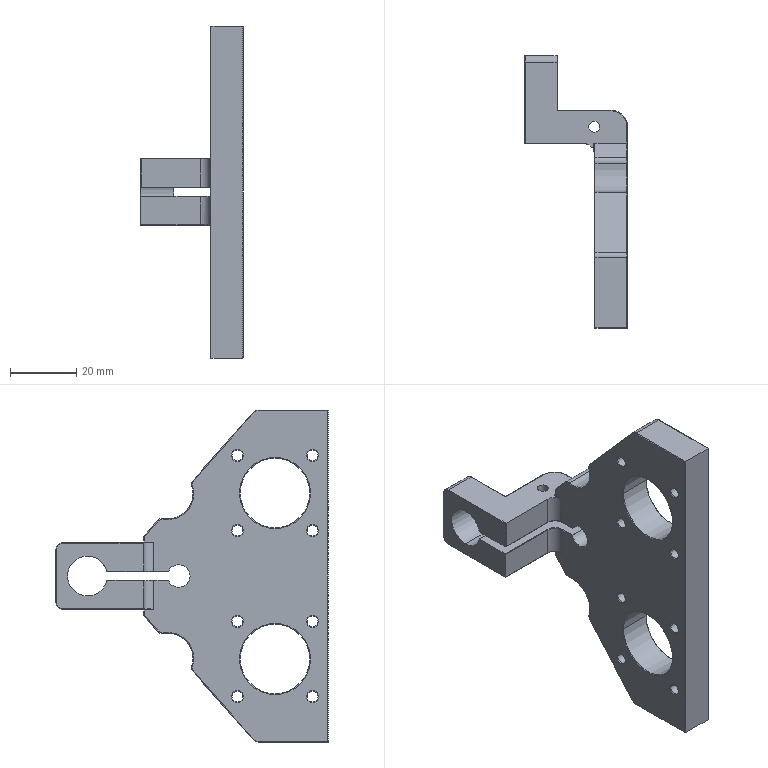Component | SolidWorks | NozzleFixingPlate-1 | 1 solid | 201 faces | volume 40915 mm3 | cylinder 93 | torus 73 | plane 25 | spline 7 | cone 2 | sphere 1 | commonest cylinder face diameters 0.4 x47 3.3 x18 4 x10 21 x4 12 x3 7 x2 4.5 x2 15 x2